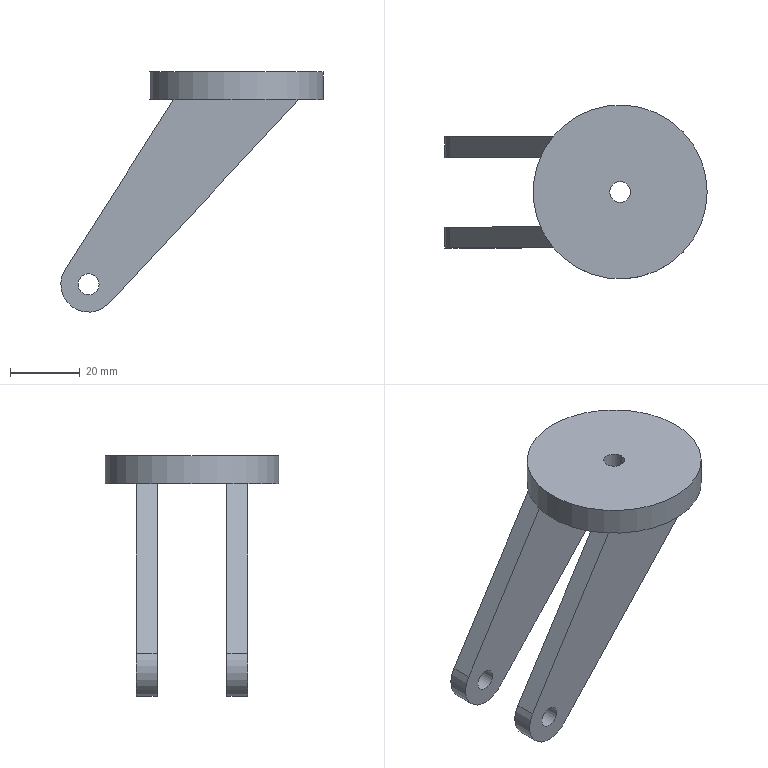Component | NX | UNI_WHEEL_CONN_FRAME | 1 solid | 16 faces | box 75.39 x 50 x 69.05 mm | volume 34354 mm3 | plane 10 | cylinder 6 | commonest cylinder face diameters 6 x3 16 x2 50 x1
STEP:
#1=CARTESIAN_POINT('',(0.,0.,0.));
#2=DIRECTION('',(0.,0.,1.));
#3=DIRECTION('',(1.,0.,0.));
#4=AXIS2_PLACEMENT_3D('',#1,#2,#3);
#5=CARTESIAN_POINT('',(447.437,-109.225,74.261));
#6=VERTEX_POINT('',#5);
#7=CARTESIAN_POINT('',(422.437,-109.225,74.261));
#8=DIRECTION('',(0.,0.,1.));
#9=DIRECTION('',(1.,0.,0.));
#10=AXIS2_PLACEMENT_3D('',#7,#8,#9);
#11=CIRCLE('',#10,25.);
#12=CARTESIAN_POINT('',(422.437,-109.225,74.261));
#13=DIRECTION('',(0.,0.,-1.));
#14=DIRECTION('',(-1.,0.,0.));
#15=AXIS2_PLACEMENT_3D('',#12,#13,#14);
#16=CYLINDRICAL_SURFACE('',#15,25.);
#17=CARTESIAN_POINT('',(9.425,0.));
#18=DIRECTION('',(-1.,0.));
#19=VECTOR('',#18,1.);
#20=LINE('',#17,#19);
#21=(GEOMETRIC_REPRESENTATION_CONTEXT(2)PARAMETRIC_REPRESENTATION_CONTEXT()REPRESENTATION_CONTEXT('',''));
#22=DEFINITIONAL_REPRESENTATION('',(#20),#21);
#23=PCURVE('',#16,#22);
#24=CARTESIAN_POINT('',(422.437,-109.225,74.261));
#25=DIRECTION('',(0.,0.,1.));
#26=DIRECTION('',(1.,0.,0.));
#27=AXIS2_PLACEMENT_3D('',#24,#25,#26);
#28=PLANE('',#27);
#29=CARTESIAN_POINT('',(0.,0.));
#30=DIRECTION('',(1.,0.));
#31=AXIS2_PLACEMENT_2D('',#29,#30);
#32=CIRCLE('',#31,25.);
#33=(GEOMETRIC_REPRESENTATION_CONTEXT(2)PARAMETRIC_REPRESENTATION_CONTEXT()REPRESENTATION_CONTEXT('',''));
#34=DEFINITIONAL_REPRESENTATION('',(#32),#33);
#35=PCURVE('',#28,#34);
#36=SURFACE_CURVE('',#11,(#23,#35),.PCURVE_S1.);
#37=EDGE_CURVE('',#6,#6,#36,.T.);
#38=ORIENTED_EDGE('',*,*,#37,.F.);
#39=CARTESIAN_POINT('',(447.437,-109.225,66.261));
#40=VERTEX_POINT('',#39);
#41=CARTESIAN_POINT('',(447.437,-109.225,74.261));
#42=CARTESIAN_POINT('',(447.437,-109.225,66.261));
#43=B_SPLINE_CURVE_WITH_KNOTS('',1,(#41,#42),.UNSPECIFIED.,.F.,.F.,(2,2),(0.,8.),.PIECEWISE_BEZIER_KNOTS.);
#44=CARTESIAN_POINT('',(9.425,0.));
#45=DIRECTION('',(0.,1.));
#46=VECTOR('',#45,1.);
#47=LINE('',#44,#46);
#48=(GEOMETRIC_REPRESENTATION_CONTEXT(2)PARAMETRIC_REPRESENTATION_CONTEXT()REPRESENTATION_CONTEXT('',''));
#49=DEFINITIONAL_REPRESENTATION('',(#47),#48);
#50=PCURVE('',#16,#49);
#51=CARTESIAN_POINT('',(3.142,0.));
#52=DIRECTION('',(0.,1.));
#53=VECTOR('',#52,1.);
#54=LINE('',#51,#53);
#55=(GEOMETRIC_REPRESENTATION_CONTEXT(2)PARAMETRIC_REPRESENTATION_CONTEXT()REPRESENTATION_CONTEXT('',''));
#56=DEFINITIONAL_REPRESENTATION('',(#54),#55);
#57=PCURVE('',#16,#56);
#58=SEAM_CURVE('',#43,(#50,#57),.PCURVE_S1.);
#59=EDGE_CURVE('',#6,#40,#58,.T.);
#60=ORIENTED_EDGE('',*,*,#59,.T.);
#61=CARTESIAN_POINT('',(422.437,-109.225,66.261));
#62=DIRECTION('',(0.,0.,1.));
#63=DIRECTION('',(1.,0.,0.));
#64=AXIS2_PLACEMENT_3D('',#61,#62,#63);
#65=CIRCLE('',#64,25.);
#66=CARTESIAN_POINT('',(9.425,8.));
#67=DIRECTION('',(-1.,0.));
#68=VECTOR('',#67,1.);
#69=LINE('',#66,#68);
#70=(GEOMETRIC_REPRESENTATION_CONTEXT(2)PARAMETRIC_REPRESENTATION_CONTEXT()REPRESENTATION_CONTEXT('',''));
#71=DEFINITIONAL_REPRESENTATION('',(#69),#70);
#72=PCURVE('',#16,#71);
#73=CARTESIAN_POINT('',(422.437,-109.225,66.261));
#74=DIRECTION('',(0.,0.,1.));
#75=DIRECTION('',(1.,0.,0.));
#76=AXIS2_PLACEMENT_3D('',#73,#74,#75);
#77=PLANE('',#76);
#78=CARTESIAN_POINT('',(0.,0.));
#79=DIRECTION('',(1.,0.));
#80=AXIS2_PLACEMENT_2D('',#78,#79);
#81=CIRCLE('',#80,25.);
#82=(GEOMETRIC_REPRESENTATION_CONTEXT(2)PARAMETRIC_REPRESENTATION_CONTEXT()REPRESENTATION_CONTEXT('',''));
#83=DEFINITIONAL_REPRESENTATION('',(#81),#82);
#84=PCURVE('',#77,#83);
#85=SURFACE_CURVE('',#65,(#72,#84),.PCURVE_S1.);
#86=EDGE_CURVE('',#40,#40,#85,.T.);
#87=ORIENTED_EDGE('',*,*,#86,.T.);
#88=ORIENTED_EDGE('',*,*,#59,.F.);
#89=EDGE_LOOP('',(#38,#60,#87,#88));
#90=FACE_BOUND('',#89,.T.);
#91=ADVANCED_FACE('',(#90),#16,.T.);
#92=CARTESIAN_POINT('',(425.437,-109.225,74.261));
#93=VERTEX_POINT('',#92);
#94=CARTESIAN_POINT('',(422.437,-109.225,74.261));
#95=DIRECTION('',(0.,0.,1.));
#96=DIRECTION('',(1.,0.,0.));
#97=AXIS2_PLACEMENT_3D('',#94,#95,#96);
#98=CIRCLE('',#97,3.);
#99=CARTESIAN_POINT('',(422.437,-109.225,74.261));
#100=DIRECTION('',(0.,0.,-1.));
#101=DIRECTION('',(-1.,0.,0.));
#102=AXIS2_PLACEMENT_3D('',#99,#100,#101);
#103=CYLINDRICAL_SURFACE('',#102,3.);
#104=CARTESIAN_POINT('',(9.425,0.));
#105=DIRECTION('',(-1.,0.));
#106=VECTOR('',#105,1.);
#107=LINE('',#104,#106);
#108=(GEOMETRIC_REPRESENTATION_CONTEXT(2)PARAMETRIC_REPRESENTATION_CONTEXT()REPRESENTATION_CONTEXT('',''));
#109=DEFINITIONAL_REPRESENTATION('',(#107),#108);
#110=PCURVE('',#103,#109);
#111=CARTESIAN_POINT('',(0.,0.));
#112=DIRECTION('',(1.,0.));
#113=AXIS2_PLACEMENT_2D('',#111,#112);
#114=CIRCLE('',#113,3.);
#115=(GEOMETRIC_REPRESENTATION_CONTEXT(2)PARAMETRIC_REPRESENTATION_CONTEXT()REPRESENTATION_CONTEXT('',''));
#116=DEFINITIONAL_REPRESENTATION('',(#114),#115);
#117=PCURVE('',#28,#116);
#118=SURFACE_CURVE('',#98,(#110,#117),.PCURVE_S1.);
#119=EDGE_CURVE('',#93,#93,#118,.T.);
#120=ORIENTED_EDGE('',*,*,#119,.F.);
#121=CARTESIAN_POINT('',(425.437,-109.225,66.261));
#122=VERTEX_POINT('',#121);
#123=CARTESIAN_POINT('',(425.437,-109.225,74.261));
#124=CARTESIAN_POINT('',(425.437,-109.225,66.261));
#125=B_SPLINE_CURVE_WITH_KNOTS('',1,(#123,#124),.UNSPECIFIED.,.F.,.F.,(2,2),(0.,8.),.PIECEWISE_BEZIER_KNOTS.);
#126=CARTESIAN_POINT('',(9.425,0.));
#127=DIRECTION('',(0.,1.));
#128=VECTOR('',#127,1.);
#129=LINE('',#126,#128);
#130=(GEOMETRIC_REPRESENTATION_CONTEXT(2)PARAMETRIC_REPRESENTATION_CONTEXT()REPRESENTATION_CONTEXT('',''));
#131=DEFINITIONAL_REPRESENTATION('',(#129),#130);
#132=PCURVE('',#103,#131);
#133=CARTESIAN_POINT('',(3.142,0.));
#134=DIRECTION('',(0.,1.));
#135=VECTOR('',#134,1.);
#136=LINE('',#133,#135);
#137=(GEOMETRIC_REPRESENTATION_CONTEXT(2)PARAMETRIC_REPRESENTATION_CONTEXT()REPRESENTATION_CONTEXT('',''));
#138=DEFINITIONAL_REPRESENTATION('',(#136),#137);
#139=PCURVE('',#103,#138);
#140=SEAM_CURVE('',#125,(#132,#139),.PCURVE_S1.);
#141=EDGE_CURVE('',#93,#122,#140,.T.);
#142=ORIENTED_EDGE('',*,*,#141,.T.);
#143=CARTESIAN_POINT('',(422.437,-109.225,66.261));
#144=DIRECTION('',(0.,0.,1.));
#145=DIRECTION('',(1.,0.,0.));
#146=AXIS2_PLACEMENT_3D('',#143,#144,#145);
#147=CIRCLE('',#146,3.);
#148=CARTESIAN_POINT('',(9.425,8.));
#149=DIRECTION('',(-1.,0.));
#150=VECTOR('',#149,1.);
#151=LINE('',#148,#150);
#152=(GEOMETRIC_REPRESENTATION_CONTEXT(2)PARAMETRIC_REPRESENTATION_CONTEXT()REPRESENTATION_CONTEXT('',''));
#153=DEFINITIONAL_REPRESENTATION('',(#151),#152);
#154=PCURVE('',#103,#153);
#155=CARTESIAN_POINT('',(0.,0.));
#156=DIRECTION('',(1.,0.));
#157=AXIS2_PLACEMENT_2D('',#155,#156);
#158=CIRCLE('',#157,3.);
#159=(GEOMETRIC_REPRESENTATION_CONTEXT(2)PARAMETRIC_REPRESENTATION_CONTEXT()REPRESENTATION_CONTEXT('',''));
#160=DEFINITIONAL_REPRESENTATION('',(#158),#159);
#161=PCURVE('',#77,#160);
#162=SURFACE_CURVE('',#147,(#154,#161),.PCURVE_S1.);
#163=EDGE_CURVE('',#122,#122,#162,.T.);
#164=ORIENTED_EDGE('',*,*,#163,.T.);
#165=ORIENTED_EDGE('',*,*,#141,.F.);
#166=EDGE_LOOP('',(#120,#142,#164,#165));
#167=FACE_BOUND('',#166,.F.);
#168=ADVANCED_FACE('',(#167),#103,.F.);
#169=ORIENTED_EDGE('',*,*,#37,.T.);
#170=EDGE_LOOP('',(#169));
#171=FACE_BOUND('',#170,.T.);
#172=ORIENTED_EDGE('',*,*,#119,.F.);
#173=EDGE_LOOP('',(#172));
#174=FACE_BOUND('',#173,.T.);
#175=ADVANCED_FACE('',(#171,#174),#28,.T.);
#176=CARTESIAN_POINT('',(440.437,-93.225,66.261));
#177=VERTEX_POINT('',#176);
#178=CARTESIAN_POINT('',(440.437,-99.225,66.261));
#179=VERTEX_POINT('',#178);
#180=CARTESIAN_POINT('',(440.437,-93.225,66.261));
#181=DIRECTION('',(0.,-1.,0.));
#182=VECTOR('',#181,1.);
#183=LINE('',#180,#182);
#184=CARTESIAN_POINT('',(18.,16.));
#185=DIRECTION('',(0.,-1.));
#186=VECTOR('',#185,1.);
#187=LINE('',#184,#186);
#188=(GEOMETRIC_REPRESENTATION_CONTEXT(2)PARAMETRIC_REPRESENTATION_CONTEXT()REPRESENTATION_CONTEXT('',''));
#189=DEFINITIONAL_REPRESENTATION('',(#187),#188);
#190=PCURVE('',#77,#189);
#191=CARTESIAN_POINT('',(385.896,-93.225,7.753));
#192=DIRECTION('',(0.7315,0.,-0.6819));
#193=DIRECTION('',(-0.6819,0.,-0.7315));
#194=AXIS2_PLACEMENT_3D('',#191,#192,#193);
#195=PLANE('',#194);
#196=CARTESIAN_POINT('',(-79.987,0.));
#197=DIRECTION('',(0.,-1.));
#198=VECTOR('',#197,1.);
#199=LINE('',#196,#198);
#200=(GEOMETRIC_REPRESENTATION_CONTEXT(2)PARAMETRIC_REPRESENTATION_CONTEXT()REPRESENTATION_CONTEXT('',''));
#201=DEFINITIONAL_REPRESENTATION('',(#199),#200);
#202=PCURVE('',#195,#201);
#203=SURFACE_CURVE('',#183,(#190,#202),.PCURVE_S1.);
#204=EDGE_CURVE('',#177,#179,#203,.T.);
#205=ORIENTED_EDGE('',*,*,#204,.F.);
#206=CARTESIAN_POINT('',(404.437,-93.225,66.261));
#207=VERTEX_POINT('',#206);
#208=CARTESIAN_POINT('',(440.437,-93.225,66.261));
#209=DIRECTION('',(-1.,0.,-0.));
#210=VECTOR('',#209,1.);
#211=LINE('',#208,#210);
#212=CARTESIAN_POINT('',(18.,16.));
#213=DIRECTION('',(-1.,0.));
#214=VECTOR('',#213,1.);
#215=LINE('',#212,#214);
#216=(GEOMETRIC_REPRESENTATION_CONTEXT(2)PARAMETRIC_REPRESENTATION_CONTEXT()REPRESENTATION_CONTEXT('',''));
#217=DEFINITIONAL_REPRESENTATION('',(#215),#216);
#218=PCURVE('',#77,#217);
#219=CARTESIAN_POINT('',(380.045,-93.225,13.208));
#220=DIRECTION('',(0.,-1.,0.));
#221=DIRECTION('',(0.,0.,-1.));
#222=AXIS2_PLACEMENT_3D('',#219,#220,#221);
#223=PLANE('',#222);
#224=CARTESIAN_POINT('',(-53.054,60.392));
#225=DIRECTION('',(0.,-1.));
#226=VECTOR('',#225,1.);
#227=LINE('',#224,#226);
#228=(GEOMETRIC_REPRESENTATION_CONTEXT(2)PARAMETRIC_REPRESENTATION_CONTEXT()REPRESENTATION_CONTEXT('',''));
#229=DEFINITIONAL_REPRESENTATION('',(#227),#228);
#230=PCURVE('',#223,#229);
#231=SURFACE_CURVE('',#211,(#218,#230),.PCURVE_S1.);
#232=EDGE_CURVE('',#177,#207,#231,.T.);
#233=ORIENTED_EDGE('',*,*,#232,.T.);
#234=CARTESIAN_POINT('',(404.437,-99.225,66.261));
#235=VERTEX_POINT('',#234);
#236=CARTESIAN_POINT('',(404.437,-93.225,66.261));
#237=DIRECTION('',(0.,-1.,0.));
#238=VECTOR('',#237,1.);
#239=LINE('',#236,#238);
#240=CARTESIAN_POINT('',(-18.,16.));
#241=DIRECTION('',(0.,-1.));
#242=VECTOR('',#241,1.);
#243=LINE('',#240,#242);
#244=(GEOMETRIC_REPRESENTATION_CONTEXT(2)PARAMETRIC_REPRESENTATION_CONTEXT()REPRESENTATION_CONTEXT('',''));
#245=DEFINITIONAL_REPRESENTATION('',(#243),#244);
#246=PCURVE('',#77,#245);
#247=CARTESIAN_POINT('',(404.437,-93.225,66.261));
#248=DIRECTION('',(-0.8428,0.,0.5383));
#249=DIRECTION('',(0.5383,0.,0.8428));
#250=AXIS2_PLACEMENT_3D('',#247,#248,#249);
#251=PLANE('',#250);
#252=CARTESIAN_POINT('',(0.,0.));
#253=DIRECTION('',(0.,-1.));
#254=VECTOR('',#253,1.);
#255=LINE('',#252,#254);
#256=(GEOMETRIC_REPRESENTATION_CONTEXT(2)PARAMETRIC_REPRESENTATION_CONTEXT()REPRESENTATION_CONTEXT('',''));
#257=DEFINITIONAL_REPRESENTATION('',(#255),#256);
#258=PCURVE('',#251,#257);
#259=SURFACE_CURVE('',#239,(#246,#258),.PCURVE_S1.);
#260=EDGE_CURVE('',#207,#235,#259,.T.);
#261=ORIENTED_EDGE('',*,*,#260,.T.);
#262=CARTESIAN_POINT('',(440.437,-99.225,66.261));
#263=DIRECTION('',(-1.,0.,-0.));
#264=VECTOR('',#263,1.);
#265=LINE('',#262,#264);
#266=CARTESIAN_POINT('',(18.,10.));
#267=DIRECTION('',(-1.,0.));
#268=VECTOR('',#267,1.);
#269=LINE('',#266,#268);
#270=(GEOMETRIC_REPRESENTATION_CONTEXT(2)PARAMETRIC_REPRESENTATION_CONTEXT()REPRESENTATION_CONTEXT('',''));
#271=DEFINITIONAL_REPRESENTATION('',(#269),#270);
#272=PCURVE('',#77,#271);
#273=CARTESIAN_POINT('',(380.045,-99.225,13.208));
#274=DIRECTION('',(0.,-1.,0.));
#275=DIRECTION('',(0.,0.,-1.));
#276=AXIS2_PLACEMENT_3D('',#273,#274,#275);
#277=PLANE('',#276);
#278=CARTESIAN_POINT('',(-53.054,60.392));
#279=DIRECTION('',(0.,-1.));
#280=VECTOR('',#279,1.);
#281=LINE('',#278,#280);
#282=(GEOMETRIC_REPRESENTATION_CONTEXT(2)PARAMETRIC_REPRESENTATION_CONTEXT()REPRESENTATION_CONTEXT('',''));
#283=DEFINITIONAL_REPRESENTATION('',(#281),#282);
#284=PCURVE('',#277,#283);
#285=SURFACE_CURVE('',#265,(#272,#284),.PCURVE_S1.);
#286=EDGE_CURVE('',#179,#235,#285,.T.);
#287=ORIENTED_EDGE('',*,*,#286,.F.);
#288=EDGE_LOOP('',(#205,#233,#261,#287));
#289=FACE_BOUND('',#288,.T.);
#290=CARTESIAN_POINT('',(440.437,-125.225,66.261));
#291=VERTEX_POINT('',#290);
#292=CARTESIAN_POINT('',(440.437,-119.225,66.261));
#293=VERTEX_POINT('',#292);
#294=CARTESIAN_POINT('',(440.437,-125.225,66.261));
#295=DIRECTION('',(0.,1.,0.));
#296=VECTOR('',#295,1.);
#297=LINE('',#294,#296);
#298=CARTESIAN_POINT('',(18.,-16.));
#299=DIRECTION('',(0.,1.));
#300=VECTOR('',#299,1.);
#301=LINE('',#298,#300);
#302=(GEOMETRIC_REPRESENTATION_CONTEXT(2)PARAMETRIC_REPRESENTATION_CONTEXT()REPRESENTATION_CONTEXT('',''));
#303=DEFINITIONAL_REPRESENTATION('',(#301),#302);
#304=PCURVE('',#77,#303);
#305=CARTESIAN_POINT('',(385.896,-125.225,7.753));
#306=DIRECTION('',(-0.7315,0.,0.6819));
#307=DIRECTION('',(0.6819,0.,0.7315));
#308=AXIS2_PLACEMENT_3D('',#305,#306,#307);
#309=PLANE('',#308);
#310=CARTESIAN_POINT('',(79.987,0.));
#311=DIRECTION('',(0.,1.));
#312=VECTOR('',#311,1.);
#313=LINE('',#310,#312);
#314=(GEOMETRIC_REPRESENTATION_CONTEXT(2)PARAMETRIC_REPRESENTATION_CONTEXT()REPRESENTATION_CONTEXT('',''));
#315=DEFINITIONAL_REPRESENTATION('',(#313),#314);
#316=PCURVE('',#309,#315);
#317=SURFACE_CURVE('',#297,(#304,#316),.PCURVE_S1.);
#318=EDGE_CURVE('',#291,#293,#317,.T.);
#319=ORIENTED_EDGE('',*,*,#318,.T.);
#320=CARTESIAN_POINT('',(404.437,-119.225,66.261));
#321=VERTEX_POINT('',#320);
#322=CARTESIAN_POINT('',(440.437,-119.225,66.261));
#323=DIRECTION('',(-1.,0.,-0.));
#324=VECTOR('',#323,1.);
#325=LINE('',#322,#324);
#326=CARTESIAN_POINT('',(18.,-10.));
#327=DIRECTION('',(-1.,0.));
#328=VECTOR('',#327,1.);
#329=LINE('',#326,#328);
#330=(GEOMETRIC_REPRESENTATION_CONTEXT(2)PARAMETRIC_REPRESENTATION_CONTEXT()REPRESENTATION_CONTEXT('',''));
#331=DEFINITIONAL_REPRESENTATION('',(#329),#330);
#332=PCURVE('',#77,#331);
#333=CARTESIAN_POINT('',(380.045,-119.225,13.208));
#334=DIRECTION('',(0.,-1.,0.));
#335=DIRECTION('',(0.,0.,-1.));
#336=AXIS2_PLACEMENT_3D('',#333,#334,#335);
#337=PLANE('',#336);
#338=CARTESIAN_POINT('',(-53.054,60.392));
#339=DIRECTION('',(0.,-1.));
#340=VECTOR('',#339,1.);
#341=LINE('',#338,#340);
#342=(GEOMETRIC_REPRESENTATION_CONTEXT(2)PARAMETRIC_REPRESENTATION_CONTEXT()REPRESENTATION_CONTEXT('',''));
#343=DEFINITIONAL_REPRESENTATION('',(#341),#342);
#344=PCURVE('',#337,#343);
#345=SURFACE_CURVE('',#325,(#332,#344),.PCURVE_S1.);
#346=EDGE_CURVE('',#293,#321,#345,.T.);
#347=ORIENTED_EDGE('',*,*,#346,.T.);
#348=CARTESIAN_POINT('',(404.437,-125.225,66.261));
#349=VERTEX_POINT('',#348);
#350=CARTESIAN_POINT('',(404.437,-125.225,66.261));
#351=DIRECTION('',(0.,1.,0.));
#352=VECTOR('',#351,1.);
#353=LINE('',#350,#352);
#354=CARTESIAN_POINT('',(-18.,-16.));
#355=DIRECTION('',(0.,1.));
#356=VECTOR('',#355,1.);
#357=LINE('',#354,#356);
#358=(GEOMETRIC_REPRESENTATION_CONTEXT(2)PARAMETRIC_REPRESENTATION_CONTEXT()REPRESENTATION_CONTEXT('',''));
#359=DEFINITIONAL_REPRESENTATION('',(#357),#358);
#360=PCURVE('',#77,#359);
#361=CARTESIAN_POINT('',(404.437,-125.225,66.261));
#362=DIRECTION('',(0.8428,0.,-0.5383));
#363=DIRECTION('',(-0.5383,0.,-0.8428));
#364=AXIS2_PLACEMENT_3D('',#361,#362,#363);
#365=PLANE('',#364);
#366=CARTESIAN_POINT('',(0.,0.));
#367=DIRECTION('',(0.,1.));
#368=VECTOR('',#367,1.);
#369=LINE('',#366,#368);
#370=(GEOMETRIC_REPRESENTATION_CONTEXT(2)PARAMETRIC_REPRESENTATION_CONTEXT()REPRESENTATION_CONTEXT('',''));
#371=DEFINITIONAL_REPRESENTATION('',(#369),#370);
#372=PCURVE('',#365,#371);
#373=SURFACE_CURVE('',#353,(#360,#372),.PCURVE_S1.);
#374=EDGE_CURVE('',#349,#321,#373,.T.);
#375=ORIENTED_EDGE('',*,*,#374,.F.);
#376=CARTESIAN_POINT('',(440.437,-125.225,66.261));
#377=DIRECTION('',(-1.,0.,-0.));
#378=VECTOR('',#377,1.);
#379=LINE('',#376,#378);
#380=CARTESIAN_POINT('',(18.,-16.));
#381=DIRECTION('',(-1.,0.));
#382=VECTOR('',#381,1.);
#383=LINE('',#380,#382);
#384=(GEOMETRIC_REPRESENTATION_CONTEXT(2)PARAMETRIC_REPRESENTATION_CONTEXT()REPRESENTATION_CONTEXT('',''));
#385=DEFINITIONAL_REPRESENTATION('',(#383),#384);
#386=PCURVE('',#77,#385);
#387=CARTESIAN_POINT('',(380.045,-125.225,13.208));
#388=DIRECTION('',(0.,-1.,0.));
#389=DIRECTION('',(0.,0.,-1.));
#390=AXIS2_PLACEMENT_3D('',#387,#388,#389);
#391=PLANE('',#390);
#392=CARTESIAN_POINT('',(-53.054,60.392));
#393=DIRECTION('',(0.,-1.));
#394=VECTOR('',#393,1.);
#395=LINE('',#392,#394);
#396=(GEOMETRIC_REPRESENTATION_CONTEXT(2)PARAMETRIC_REPRESENTATION_CONTEXT()REPRESENTATION_CONTEXT('',''));
#397=DEFINITIONAL_REPRESENTATION('',(#395),#396);
#398=PCURVE('',#391,#397);
#399=SURFACE_CURVE('',#379,(#386,#398),.PCURVE_S1.);
#400=EDGE_CURVE('',#291,#349,#399,.T.);
#401=ORIENTED_EDGE('',*,*,#400,.F.);
#402=EDGE_LOOP('',(#319,#347,#375,#401));
#403=FACE_BOUND('',#402,.T.);
#404=ORIENTED_EDGE('',*,*,#86,.F.);
#405=EDGE_LOOP('',(#404));
#406=FACE_BOUND('',#405,.T.);
#407=ORIENTED_EDGE('',*,*,#163,.T.);
#408=EDGE_LOOP('',(#407));
#409=FACE_BOUND('',#408,.T.);
#410=ADVANCED_FACE('',(#289,#403,#406,#409),#77,.F.);
#411=CARTESIAN_POINT('',(373.302,-119.225,17.514));
#412=VERTEX_POINT('',#411);
#413=CARTESIAN_POINT('',(385.896,-119.225,7.753));
#414=VERTEX_POINT('',#413);
#415=CARTESIAN_POINT('',(380.045,-119.225,13.208));
#416=DIRECTION('',(0.,-1.,0.));
#417=DIRECTION('',(1.,0.,0.));
#418=AXIS2_PLACEMENT_3D('',#415,#416,#417);
#419=CIRCLE('',#418,8.);
#420=CARTESIAN_POINT('',(380.045,-125.225,13.208));
#421=DIRECTION('',(0.,1.,0.));
#422=DIRECTION('',(0.,0.,1.));
#423=AXIS2_PLACEMENT_3D('',#420,#421,#422);
#424=CYLINDRICAL_SURFACE('',#423,8.);
#425=CARTESIAN_POINT('',(7.854,6.));
#426=DIRECTION('',(-1.,0.));
#427=VECTOR('',#426,1.);
#428=LINE('',#425,#427);
#429=(GEOMETRIC_REPRESENTATION_CONTEXT(2)PARAMETRIC_REPRESENTATION_CONTEXT()REPRESENTATION_CONTEXT('',''));
#430=DEFINITIONAL_REPRESENTATION('',(#428),#429);
#431=PCURVE('',#424,#430);
#432=CARTESIAN_POINT('',(0.,0.));
#433=DIRECTION('',(0.,1.));
#434=AXIS2_PLACEMENT_2D('',#432,#433);
#435=CIRCLE('',#434,8.);
#436=(GEOMETRIC_REPRESENTATION_CONTEXT(2)PARAMETRIC_REPRESENTATION_CONTEXT()REPRESENTATION_CONTEXT('',''));
#437=DEFINITIONAL_REPRESENTATION('',(#435),#436);
#438=PCURVE('',#337,#437);
#439=SURFACE_CURVE('',#419,(#431,#438),.PCURVE_S1.);
#440=EDGE_CURVE('',#412,#414,#439,.T.);
#441=ORIENTED_EDGE('',*,*,#440,.T.);
#442=CARTESIAN_POINT('',(385.896,-125.225,7.753));
#443=VERTEX_POINT('',#442);
#444=CARTESIAN_POINT('',(385.896,-125.225,7.753));
#445=DIRECTION('',(0.,1.,0.));
#446=VECTOR('',#445,1.);
#447=LINE('',#444,#446);
#448=CARTESIAN_POINT('',(2.321,0.));
#449=DIRECTION('',(0.,1.));
#450=VECTOR('',#449,1.);
#451=LINE('',#448,#450);
#452=(GEOMETRIC_REPRESENTATION_CONTEXT(2)PARAMETRIC_REPRESENTATION_CONTEXT()REPRESENTATION_CONTEXT('',''));
#453=DEFINITIONAL_REPRESENTATION('',(#451),#452);
#454=PCURVE('',#424,#453);
#455=CARTESIAN_POINT('',(-0.,0.));
#456=DIRECTION('',(0.,1.));
#457=VECTOR('',#456,1.);
#458=LINE('',#455,#457);
#459=(GEOMETRIC_REPRESENTATION_CONTEXT(2)PARAMETRIC_REPRESENTATION_CONTEXT()REPRESENTATION_CONTEXT('',''));
#460=DEFINITIONAL_REPRESENTATION('',(#458),#459);
#461=PCURVE('',#309,#460);
#462=SURFACE_CURVE('',#447,(#454,#461),.PCURVE_S1.);
#463=EDGE_CURVE('',#443,#414,#462,.T.);
#464=ORIENTED_EDGE('',*,*,#463,.F.);
#465=CARTESIAN_POINT('',(373.302,-125.225,17.514));
#466=VERTEX_POINT('',#465);
#467=CARTESIAN_POINT('',(380.045,-125.225,13.208));
#468=DIRECTION('',(0.,-1.,0.));
#469=DIRECTION('',(1.,0.,0.));
#470=AXIS2_PLACEMENT_3D('',#467,#468,#469);
#471=CIRCLE('',#470,8.);
#472=CARTESIAN_POINT('',(7.854,0.));
#473=DIRECTION('',(-1.,0.));
#474=VECTOR('',#473,1.);
#475=LINE('',#472,#474);
#476=(GEOMETRIC_REPRESENTATION_CONTEXT(2)PARAMETRIC_REPRESENTATION_CONTEXT()REPRESENTATION_CONTEXT('',''));
#477=DEFINITIONAL_REPRESENTATION('',(#475),#476);
#478=PCURVE('',#424,#477);
#479=CARTESIAN_POINT('',(0.,0.));
#480=DIRECTION('',(0.,1.));
#481=AXIS2_PLACEMENT_2D('',#479,#480);
#482=CIRCLE('',#481,8.);
#483=(GEOMETRIC_REPRESENTATION_CONTEXT(2)PARAMETRIC_REPRESENTATION_CONTEXT()REPRESENTATION_CONTEXT('',''));
#484=DEFINITIONAL_REPRESENTATION('',(#482),#483);
#485=PCURVE('',#391,#484);
#486=SURFACE_CURVE('',#471,(#478,#485),.PCURVE_S1.);
#487=EDGE_CURVE('',#466,#443,#486,.T.);
#488=ORIENTED_EDGE('',*,*,#487,.F.);
#489=CARTESIAN_POINT('',(373.302,-125.225,17.514));
#490=DIRECTION('',(0.,1.,0.));
#491=VECTOR('',#490,1.);
#492=LINE('',#489,#491);
#493=CARTESIAN_POINT('',(5.281,0.));
#494=DIRECTION('',(0.,1.));
#495=VECTOR('',#494,1.);
#496=LINE('',#493,#495);
#497=(GEOMETRIC_REPRESENTATION_CONTEXT(2)PARAMETRIC_REPRESENTATION_CONTEXT()REPRESENTATION_CONTEXT('',''));
#498=DEFINITIONAL_REPRESENTATION('',(#496),#497);
#499=PCURVE('',#424,#498);
#500=CARTESIAN_POINT('',(57.842,0.));
#501=DIRECTION('',(0.,1.));
#502=VECTOR('',#501,1.);
#503=LINE('',#500,#502);
#504=(GEOMETRIC_REPRESENTATION_CONTEXT(2)PARAMETRIC_REPRESENTATION_CONTEXT()REPRESENTATION_CONTEXT('',''));
#505=DEFINITIONAL_REPRESENTATION('',(#503),#504);
#506=PCURVE('',#365,#505);
#507=SURFACE_CURVE('',#492,(#499,#506),.PCURVE_S1.);
#508=EDGE_CURVE('',#466,#412,#507,.T.);
#509=ORIENTED_EDGE('',*,*,#508,.T.);
#510=EDGE_LOOP('',(#441,#464,#488,#509));
#511=FACE_BOUND('',#510,.T.);
#512=ADVANCED_FACE('',(#511),#424,.T.);
#513=CARTESIAN_POINT('',(385.896,-119.225,7.753));
#514=DIRECTION('',(0.6819,0.,0.7315));
#515=VECTOR('',#514,1.);
#516=LINE('',#513,#515);
#517=CARTESIAN_POINT('',(0.,6.));
#518=DIRECTION('',(1.,0.));
#519=VECTOR('',#518,1.);
#520=LINE('',#517,#519);
#521=(GEOMETRIC_REPRESENTATION_CONTEXT(2)PARAMETRIC_REPRESENTATION_CONTEXT()REPRESENTATION_CONTEXT('',''));
#522=DEFINITIONAL_REPRESENTATION('',(#520),#521);
#523=PCURVE('',#309,#522);
#524=CARTESIAN_POINT('',(5.455,5.852));
#525=DIRECTION('',(-0.7315,0.6819));
#526=VECTOR('',#525,1.);
#527=LINE('',#524,#526);
#528=(GEOMETRIC_REPRESENTATION_CONTEXT(2)PARAMETRIC_REPRESENTATION_CONTEXT()REPRESENTATION_CONTEXT('',''));
#529=DEFINITIONAL_REPRESENTATION('',(#527),#528);
#530=PCURVE('',#337,#529);
#531=SURFACE_CURVE('',#516,(#523,#530),.PCURVE_S1.);
#532=EDGE_CURVE('',#414,#293,#531,.T.);
#533=ORIENTED_EDGE('',*,*,#532,.T.);
#534=ORIENTED_EDGE('',*,*,#318,.F.);
#535=CARTESIAN_POINT('',(385.896,-125.225,7.753));
#536=DIRECTION('',(0.6819,0.,0.7315));
#537=VECTOR('',#536,1.);
#538=LINE('',#535,#537);
#539=CARTESIAN_POINT('',(0.,0.));
#540=DIRECTION('',(1.,0.));
#541=VECTOR('',#540,1.);
#542=LINE('',#539,#541);
#543=(GEOMETRIC_REPRESENTATION_CONTEXT(2)PARAMETRIC_REPRESENTATION_CONTEXT()REPRESENTATION_CONTEXT('',''));
#544=DEFINITIONAL_REPRESENTATION('',(#542),#543);
#545=PCURVE('',#309,#544);
#546=CARTESIAN_POINT('',(5.455,5.852));
#547=DIRECTION('',(-0.7315,0.6819));
#548=VECTOR('',#547,1.);
#549=LINE('',#546,#548);
#550=(GEOMETRIC_REPRESENTATION_CONTEXT(2)PARAMETRIC_REPRESENTATION_CONTEXT()REPRESENTATION_CONTEXT('',''));
#551=DEFINITIONAL_REPRESENTATION('',(#549),#550);
#552=PCURVE('',#391,#551);
#553=SURFACE_CURVE('',#538,(#545,#552),.PCURVE_S1.);
#554=EDGE_CURVE('',#443,#291,#553,.T.);
#555=ORIENTED_EDGE('',*,*,#554,.F.);
#556=ORIENTED_EDGE('',*,*,#463,.T.);
#557=EDGE_LOOP('',(#533,#534,#555,#556));
#558=FACE_BOUND('',#557,.T.);
#559=ADVANCED_FACE('',(#558),#309,.F.);
#560=CARTESIAN_POINT('',(404.437,-119.225,66.261));
#561=DIRECTION('',(-0.5383,0.,-0.8428));
#562=VECTOR('',#561,1.);
#563=LINE('',#560,#562);
#564=CARTESIAN_POINT('',(0.,6.));
#565=DIRECTION('',(1.,0.));
#566=VECTOR('',#565,1.);
#567=LINE('',#564,#566);
#568=(GEOMETRIC_REPRESENTATION_CONTEXT(2)PARAMETRIC_REPRESENTATION_CONTEXT()REPRESENTATION_CONTEXT('',''));
#569=DEFINITIONAL_REPRESENTATION('',(#567),#568);
#570=PCURVE('',#365,#569);
#571=CARTESIAN_POINT('',(-53.054,24.392));
#572=DIRECTION('',(0.8428,-0.5383));
#573=VECTOR('',#572,1.);
#574=LINE('',#571,#573);
#575=(GEOMETRIC_REPRESENTATION_CONTEXT(2)PARAMETRIC_REPRESENTATION_CONTEXT()REPRESENTATION_CONTEXT('',''));
#576=DEFINITIONAL_REPRESENTATION('',(#574),#575);
#577=PCURVE('',#337,#576);
#578=SURFACE_CURVE('',#563,(#570,#577),.PCURVE_S1.);
#579=EDGE_CURVE('',#321,#412,#578,.T.);
#580=ORIENTED_EDGE('',*,*,#579,.T.);
#581=ORIENTED_EDGE('',*,*,#508,.F.);
#582=CARTESIAN_POINT('',(404.437,-125.225,66.261));
#583=DIRECTION('',(-0.5383,0.,-0.8428));
#584=VECTOR('',#583,1.);
#585=LINE('',#582,#584);
#586=CARTESIAN_POINT('',(0.,0.));
#587=DIRECTION('',(1.,0.));
#588=VECTOR('',#587,1.);
#589=LINE('',#586,#588);
#590=(GEOMETRIC_REPRESENTATION_CONTEXT(2)PARAMETRIC_REPRESENTATION_CONTEXT()REPRESENTATION_CONTEXT('',''));
#591=DEFINITIONAL_REPRESENTATION('',(#589),#590);
#592=PCURVE('',#365,#591);
#593=CARTESIAN_POINT('',(-53.054,24.392));
#594=DIRECTION('',(0.8428,-0.5383));
#595=VECTOR('',#594,1.);
#596=LINE('',#593,#595);
#597=(GEOMETRIC_REPRESENTATION_CONTEXT(2)PARAMETRIC_REPRESENTATION_CONTEXT()REPRESENTATION_CONTEXT('',''));
#598=DEFINITIONAL_REPRESENTATION('',(#596),#597);
#599=PCURVE('',#391,#598);
#600=SURFACE_CURVE('',#585,(#592,#599),.PCURVE_S1.);
#601=EDGE_CURVE('',#349,#466,#600,.T.);
#602=ORIENTED_EDGE('',*,*,#601,.F.);
#603=ORIENTED_EDGE('',*,*,#374,.T.);
#604=EDGE_LOOP('',(#580,#581,#602,#603));
#605=FACE_BOUND('',#604,.T.);
#606=ADVANCED_FACE('',(#605),#365,.F.);
#607=CARTESIAN_POINT('',(383.045,-125.225,13.208));
#608=VERTEX_POINT('',#607);
#609=CARTESIAN_POINT('',(380.045,-125.225,13.208));
#610=DIRECTION('',(0.,-1.,0.));
#611=DIRECTION('',(1.,0.,0.));
#612=AXIS2_PLACEMENT_3D('',#609,#610,#611);
#613=CIRCLE('',#612,3.);
#614=CARTESIAN_POINT('',(380.045,-125.225,13.208));
#615=DIRECTION('',(0.,1.,0.));
#616=DIRECTION('',(0.,0.,1.));
#617=AXIS2_PLACEMENT_3D('',#614,#615,#616);
#618=CYLINDRICAL_SURFACE('',#617,3.);
#619=CARTESIAN_POINT('',(7.854,0.));
#620=DIRECTION('',(-1.,0.));
#621=VECTOR('',#620,1.);
#622=LINE('',#619,#621);
#623=(GEOMETRIC_REPRESENTATION_CONTEXT(2)PARAMETRIC_REPRESENTATION_CONTEXT()REPRESENTATION_CONTEXT('',''));
#624=DEFINITIONAL_REPRESENTATION('',(#622),#623);
#625=PCURVE('',#618,#624);
#626=CARTESIAN_POINT('',(0.,0.));
#627=DIRECTION('',(0.,1.));
#628=AXIS2_PLACEMENT_2D('',#626,#627);
#629=CIRCLE('',#628,3.);
#630=(GEOMETRIC_REPRESENTATION_CONTEXT(2)PARAMETRIC_REPRESENTATION_CONTEXT()REPRESENTATION_CONTEXT('',''));
#631=DEFINITIONAL_REPRESENTATION('',(#629),#630);
#632=PCURVE('',#391,#631);
#633=SURFACE_CURVE('',#613,(#625,#632),.PCURVE_S1.);
#634=EDGE_CURVE('',#608,#608,#633,.T.);
#635=ORIENTED_EDGE('',*,*,#634,.F.);
#636=CARTESIAN_POINT('',(383.045,-119.225,13.208));
#637=VERTEX_POINT('',#636);
#638=CARTESIAN_POINT('',(383.045,-125.225,13.208));
#639=CARTESIAN_POINT('',(383.045,-119.225,13.208));
#640=B_SPLINE_CURVE_WITH_KNOTS('',1,(#638,#639),.UNSPECIFIED.,.F.,.F.,(2,2),(0.,6.),.PIECEWISE_BEZIER_KNOTS.);
#641=CARTESIAN_POINT('',(7.854,0.));
#642=DIRECTION('',(0.,1.));
#643=VECTOR('',#642,1.);
#644=LINE('',#641,#643);
#645=(GEOMETRIC_REPRESENTATION_CONTEXT(2)PARAMETRIC_REPRESENTATION_CONTEXT()REPRESENTATION_CONTEXT('',''));
#646=DEFINITIONAL_REPRESENTATION('',(#644),#645);
#647=PCURVE('',#618,#646);
#648=CARTESIAN_POINT('',(1.571,0.));
#649=DIRECTION('',(0.,1.));
#650=VECTOR('',#649,1.);
#651=LINE('',#648,#650);
#652=(GEOMETRIC_REPRESENTATION_CONTEXT(2)PARAMETRIC_REPRESENTATION_CONTEXT()REPRESENTATION_CONTEXT('',''));
#653=DEFINITIONAL_REPRESENTATION('',(#651),#652);
#654=PCURVE('',#618,#653);
#655=SEAM_CURVE('',#640,(#647,#654),.PCURVE_S1.);
#656=EDGE_CURVE('',#608,#637,#655,.T.);
#657=ORIENTED_EDGE('',*,*,#656,.T.);
#658=CARTESIAN_POINT('',(380.045,-119.225,13.208));
#659=DIRECTION('',(0.,-1.,0.));
#660=DIRECTION('',(1.,0.,0.));
#661=AXIS2_PLACEMENT_3D('',#658,#659,#660);
#662=CIRCLE('',#661,3.);
#663=CARTESIAN_POINT('',(7.854,6.));
#664=DIRECTION('',(-1.,0.));
#665=VECTOR('',#664,1.);
#666=LINE('',#663,#665);
#667=(GEOMETRIC_REPRESENTATION_CONTEXT(2)PARAMETRIC_REPRESENTATION_CONTEXT()REPRESENTATION_CONTEXT('',''));
#668=DEFINITIONAL_REPRESENTATION('',(#666),#667);
#669=PCURVE('',#618,#668);
#670=CARTESIAN_POINT('',(0.,0.));
#671=DIRECTION('',(0.,1.));
#672=AXIS2_PLACEMENT_2D('',#670,#671);
#673=CIRCLE('',#672,3.);
#674=(GEOMETRIC_REPRESENTATION_CONTEXT(2)PARAMETRIC_REPRESENTATION_CONTEXT()REPRESENTATION_CONTEXT('',''));
#675=DEFINITIONAL_REPRESENTATION('',(#673),#674);
#676=PCURVE('',#337,#675);
#677=SURFACE_CURVE('',#662,(#669,#676),.PCURVE_S1.);
#678=EDGE_CURVE('',#637,#637,#677,.T.);
#679=ORIENTED_EDGE('',*,*,#678,.T.);
#680=ORIENTED_EDGE('',*,*,#656,.F.);
#681=EDGE_LOOP('',(#635,#657,#679,#680));
#682=FACE_BOUND('',#681,.F.);
#683=ADVANCED_FACE('',(#682),#618,.F.);
#684=ORIENTED_EDGE('',*,*,#487,.T.);
#685=ORIENTED_EDGE('',*,*,#554,.T.);
#686=ORIENTED_EDGE('',*,*,#400,.T.);
#687=ORIENTED_EDGE('',*,*,#601,.T.);
#688=EDGE_LOOP('',(#684,#685,#686,#687));
#689=FACE_BOUND('',#688,.T.);
#690=ORIENTED_EDGE('',*,*,#634,.F.);
#691=EDGE_LOOP('',(#690));
#692=FACE_BOUND('',#691,.T.);
#693=ADVANCED_FACE('',(#689,#692),#391,.T.);
#694=ORIENTED_EDGE('',*,*,#440,.F.);
#695=ORIENTED_EDGE('',*,*,#579,.F.);
#696=ORIENTED_EDGE('',*,*,#346,.F.);
#697=ORIENTED_EDGE('',*,*,#532,.F.);
#698=EDGE_LOOP('',(#694,#695,#696,#697));
#699=FACE_BOUND('',#698,.T.);
#700=ORIENTED_EDGE('',*,*,#678,.T.);
#701=EDGE_LOOP('',(#700));
#702=FACE_BOUND('',#701,.T.);
#703=ADVANCED_FACE('',(#699,#702),#337,.F.);
#704=CARTESIAN_POINT('',(373.302,-99.225,17.514));
#705=VERTEX_POINT('',#704);
#706=CARTESIAN_POINT('',(385.896,-99.225,7.753));
#707=VERTEX_POINT('',#706);
#708=CARTESIAN_POINT('',(380.045,-99.225,13.208));
#709=DIRECTION('',(0.,-1.,0.));
#710=DIRECTION('',(1.,0.,0.));
#711=AXIS2_PLACEMENT_3D('',#708,#709,#710);
#712=CIRCLE('',#711,8.);
#713=CARTESIAN_POINT('',(380.045,-93.225,13.208));
#714=DIRECTION('',(0.,-1.,0.));
#715=DIRECTION('',(0.,0.,-1.));
#716=AXIS2_PLACEMENT_3D('',#713,#714,#715);
#717=CYLINDRICAL_SURFACE('',#716,8.);
#718=CARTESIAN_POINT('',(1.571,6.));
#719=DIRECTION('',(1.,0.));
#720=VECTOR('',#719,1.);
#721=LINE('',#718,#720);
#722=(GEOMETRIC_REPRESENTATION_CONTEXT(2)PARAMETRIC_REPRESENTATION_CONTEXT()REPRESENTATION_CONTEXT('',''));
#723=DEFINITIONAL_REPRESENTATION('',(#721),#722);
#724=PCURVE('',#717,#723);
#725=CARTESIAN_POINT('',(0.,0.));
#726=DIRECTION('',(0.,1.));
#727=AXIS2_PLACEMENT_2D('',#725,#726);
#728=CIRCLE('',#727,8.);
#729=(GEOMETRIC_REPRESENTATION_CONTEXT(2)PARAMETRIC_REPRESENTATION_CONTEXT()REPRESENTATION_CONTEXT('',''));
#730=DEFINITIONAL_REPRESENTATION('',(#728),#729);
#731=PCURVE('',#277,#730);
#732=SURFACE_CURVE('',#712,(#724,#731),.PCURVE_S1.);
#733=EDGE_CURVE('',#705,#707,#732,.T.);
#734=ORIENTED_EDGE('',*,*,#733,.F.);
#735=CARTESIAN_POINT('',(373.302,-93.225,17.514));
#736=VERTEX_POINT('',#735);
#737=CARTESIAN_POINT('',(373.302,-93.225,17.514));
#738=DIRECTION('',(0.,-1.,0.));
#739=VECTOR('',#738,1.);
#740=LINE('',#737,#739);
#741=CARTESIAN_POINT('',(4.144,0.));
#742=DIRECTION('',(0.,1.));
#743=VECTOR('',#742,1.);
#744=LINE('',#741,#743);
#745=(GEOMETRIC_REPRESENTATION_CONTEXT(2)PARAMETRIC_REPRESENTATION_CONTEXT()REPRESENTATION_CONTEXT('',''));
#746=DEFINITIONAL_REPRESENTATION('',(#744),#745);
#747=PCURVE('',#717,#746);
#748=CARTESIAN_POINT('',(-57.842,0.));
#749=DIRECTION('',(0.,-1.));
#750=VECTOR('',#749,1.);
#751=LINE('',#748,#750);
#752=(GEOMETRIC_REPRESENTATION_CONTEXT(2)PARAMETRIC_REPRESENTATION_CONTEXT()REPRESENTATION_CONTEXT('',''));
#753=DEFINITIONAL_REPRESENTATION('',(#751),#752);
#754=PCURVE('',#251,#753);
#755=SURFACE_CURVE('',#740,(#747,#754),.PCURVE_S1.);
#756=EDGE_CURVE('',#736,#705,#755,.T.);
#757=ORIENTED_EDGE('',*,*,#756,.F.);
#758=CARTESIAN_POINT('',(385.896,-93.225,7.753));
#759=VERTEX_POINT('',#758);
#760=CARTESIAN_POINT('',(380.045,-93.225,13.208));
#761=DIRECTION('',(0.,-1.,0.));
#762=DIRECTION('',(1.,0.,0.));
#763=AXIS2_PLACEMENT_3D('',#760,#761,#762);
#764=CIRCLE('',#763,8.);
#765=CARTESIAN_POINT('',(1.571,0.));
#766=DIRECTION('',(1.,0.));
#767=VECTOR('',#766,1.);
#768=LINE('',#765,#767);
#769=(GEOMETRIC_REPRESENTATION_CONTEXT(2)PARAMETRIC_REPRESENTATION_CONTEXT()REPRESENTATION_CONTEXT('',''));
#770=DEFINITIONAL_REPRESENTATION('',(#768),#769);
#771=PCURVE('',#717,#770);
#772=CARTESIAN_POINT('',(0.,0.));
#773=DIRECTION('',(0.,1.));
#774=AXIS2_PLACEMENT_2D('',#772,#773);
#775=CIRCLE('',#774,8.);
#776=(GEOMETRIC_REPRESENTATION_CONTEXT(2)PARAMETRIC_REPRESENTATION_CONTEXT()REPRESENTATION_CONTEXT('',''));
#777=DEFINITIONAL_REPRESENTATION('',(#775),#776);
#778=PCURVE('',#223,#777);
#779=SURFACE_CURVE('',#764,(#771,#778),.PCURVE_S1.);
#780=EDGE_CURVE('',#736,#759,#779,.T.);
#781=ORIENTED_EDGE('',*,*,#780,.T.);
#782=CARTESIAN_POINT('',(385.896,-93.225,7.753));
#783=DIRECTION('',(0.,-1.,0.));
#784=VECTOR('',#783,1.);
#785=LINE('',#782,#784);
#786=CARTESIAN_POINT('',(7.104,0.));
#787=DIRECTION('',(0.,1.));
#788=VECTOR('',#787,1.);
#789=LINE('',#786,#788);
#790=(GEOMETRIC_REPRESENTATION_CONTEXT(2)PARAMETRIC_REPRESENTATION_CONTEXT()REPRESENTATION_CONTEXT('',''));
#791=DEFINITIONAL_REPRESENTATION('',(#789),#790);
#792=PCURVE('',#717,#791);
#793=CARTESIAN_POINT('',(0.,0.));
#794=DIRECTION('',(0.,-1.));
#795=VECTOR('',#794,1.);
#796=LINE('',#793,#795);
#797=(GEOMETRIC_REPRESENTATION_CONTEXT(2)PARAMETRIC_REPRESENTATION_CONTEXT()REPRESENTATION_CONTEXT('',''));
#798=DEFINITIONAL_REPRESENTATION('',(#796),#797);
#799=PCURVE('',#195,#798);
#800=SURFACE_CURVE('',#785,(#792,#799),.PCURVE_S1.);
#801=EDGE_CURVE('',#759,#707,#800,.T.);
#802=ORIENTED_EDGE('',*,*,#801,.T.);
#803=EDGE_LOOP('',(#734,#757,#781,#802));
#804=FACE_BOUND('',#803,.T.);
#805=ADVANCED_FACE('',(#804),#717,.T.);
#806=CARTESIAN_POINT('',(385.896,-99.225,7.753));
#807=DIRECTION('',(0.6819,0.,0.7315));
#808=VECTOR('',#807,1.);
#809=LINE('',#806,#808);
#810=CARTESIAN_POINT('',(0.,-6.));
#811=DIRECTION('',(-1.,0.));
#812=VECTOR('',#811,1.);
#813=LINE('',#810,#812);
#814=(GEOMETRIC_REPRESENTATION_CONTEXT(2)PARAMETRIC_REPRESENTATION_CONTEXT()REPRESENTATION_CONTEXT('',''));
#815=DEFINITIONAL_REPRESENTATION('',(#813),#814);
#816=PCURVE('',#195,#815);
#817=CARTESIAN_POINT('',(5.455,5.852));
#818=DIRECTION('',(-0.7315,0.6819));
#819=VECTOR('',#818,1.);
#820=LINE('',#817,#819);
#821=(GEOMETRIC_REPRESENTATION_CONTEXT(2)PARAMETRIC_REPRESENTATION_CONTEXT()REPRESENTATION_CONTEXT('',''));
#822=DEFINITIONAL_REPRESENTATION('',(#820),#821);
#823=PCURVE('',#277,#822);
#824=SURFACE_CURVE('',#809,(#816,#823),.PCURVE_S1.);
#825=EDGE_CURVE('',#707,#179,#824,.T.);
#826=ORIENTED_EDGE('',*,*,#825,.F.);
#827=ORIENTED_EDGE('',*,*,#801,.F.);
#828=CARTESIAN_POINT('',(385.896,-93.225,7.753));
#829=DIRECTION('',(0.6819,0.,0.7315));
#830=VECTOR('',#829,1.);
#831=LINE('',#828,#830);
#832=CARTESIAN_POINT('',(0.,0.));
#833=DIRECTION('',(-1.,0.));
#834=VECTOR('',#833,1.);
#835=LINE('',#832,#834);
#836=(GEOMETRIC_REPRESENTATION_CONTEXT(2)PARAMETRIC_REPRESENTATION_CONTEXT()REPRESENTATION_CONTEXT('',''));
#837=DEFINITIONAL_REPRESENTATION('',(#835),#836);
#838=PCURVE('',#195,#837);
#839=CARTESIAN_POINT('',(5.455,5.852));
#840=DIRECTION('',(-0.7315,0.6819));
#841=VECTOR('',#840,1.);
#842=LINE('',#839,#841);
#843=(GEOMETRIC_REPRESENTATION_CONTEXT(2)PARAMETRIC_REPRESENTATION_CONTEXT()REPRESENTATION_CONTEXT('',''));
#844=DEFINITIONAL_REPRESENTATION('',(#842),#843);
#845=PCURVE('',#223,#844);
#846=SURFACE_CURVE('',#831,(#838,#845),.PCURVE_S1.);
#847=EDGE_CURVE('',#759,#177,#846,.T.);
#848=ORIENTED_EDGE('',*,*,#847,.T.);
#849=ORIENTED_EDGE('',*,*,#204,.T.);
#850=EDGE_LOOP('',(#826,#827,#848,#849));
#851=FACE_BOUND('',#850,.T.);
#852=ADVANCED_FACE('',(#851),#195,.T.);
#853=CARTESIAN_POINT('',(404.437,-99.225,66.261));
#854=DIRECTION('',(-0.5383,0.,-0.8428));
#855=VECTOR('',#854,1.);
#856=LINE('',#853,#855);
#857=CARTESIAN_POINT('',(0.,-6.));
#858=DIRECTION('',(-1.,0.));
#859=VECTOR('',#858,1.);
#860=LINE('',#857,#859);
#861=(GEOMETRIC_REPRESENTATION_CONTEXT(2)PARAMETRIC_REPRESENTATION_CONTEXT()REPRESENTATION_CONTEXT('',''));
#862=DEFINITIONAL_REPRESENTATION('',(#860),#861);
#863=PCURVE('',#251,#862);
#864=CARTESIAN_POINT('',(-53.054,24.392));
#865=DIRECTION('',(0.8428,-0.5383));
#866=VECTOR('',#865,1.);
#867=LINE('',#864,#866);
#868=(GEOMETRIC_REPRESENTATION_CONTEXT(2)PARAMETRIC_REPRESENTATION_CONTEXT()REPRESENTATION_CONTEXT('',''));
#869=DEFINITIONAL_REPRESENTATION('',(#867),#868);
#870=PCURVE('',#277,#869);
#871=SURFACE_CURVE('',#856,(#863,#870),.PCURVE_S1.);
#872=EDGE_CURVE('',#235,#705,#871,.T.);
#873=ORIENTED_EDGE('',*,*,#872,.F.);
#874=ORIENTED_EDGE('',*,*,#260,.F.);
#875=CARTESIAN_POINT('',(404.437,-93.225,66.261));
#876=DIRECTION('',(-0.5383,0.,-0.8428));
#877=VECTOR('',#876,1.);
#878=LINE('',#875,#877);
#879=CARTESIAN_POINT('',(0.,0.));
#880=DIRECTION('',(-1.,0.));
#881=VECTOR('',#880,1.);
#882=LINE('',#879,#881);
#883=(GEOMETRIC_REPRESENTATION_CONTEXT(2)PARAMETRIC_REPRESENTATION_CONTEXT()REPRESENTATION_CONTEXT('',''));
#884=DEFINITIONAL_REPRESENTATION('',(#882),#883);
#885=PCURVE('',#251,#884);
#886=CARTESIAN_POINT('',(-53.054,24.392));
#887=DIRECTION('',(0.8428,-0.5383));
#888=VECTOR('',#887,1.);
#889=LINE('',#886,#888);
#890=(GEOMETRIC_REPRESENTATION_CONTEXT(2)PARAMETRIC_REPRESENTATION_CONTEXT()REPRESENTATION_CONTEXT('',''));
#891=DEFINITIONAL_REPRESENTATION('',(#889),#890);
#892=PCURVE('',#223,#891);
#893=SURFACE_CURVE('',#878,(#885,#892),.PCURVE_S1.);
#894=EDGE_CURVE('',#207,#736,#893,.T.);
#895=ORIENTED_EDGE('',*,*,#894,.T.);
#896=ORIENTED_EDGE('',*,*,#756,.T.);
#897=EDGE_LOOP('',(#873,#874,#895,#896));
#898=FACE_BOUND('',#897,.T.);
#899=ADVANCED_FACE('',(#898),#251,.T.);
#900=CARTESIAN_POINT('',(383.045,-93.225,13.208));
#901=VERTEX_POINT('',#900);
#902=CARTESIAN_POINT('',(380.045,-93.225,13.208));
#903=DIRECTION('',(0.,-1.,0.));
#904=DIRECTION('',(1.,0.,0.));
#905=AXIS2_PLACEMENT_3D('',#902,#903,#904);
#906=CIRCLE('',#905,3.);
#907=CARTESIAN_POINT('',(380.045,-93.225,13.208));
#908=DIRECTION('',(0.,-1.,0.));
#909=DIRECTION('',(0.,0.,-1.));
#910=AXIS2_PLACEMENT_3D('',#907,#908,#909);
#911=CYLINDRICAL_SURFACE('',#910,3.);
#912=CARTESIAN_POINT('',(1.571,0.));
#913=DIRECTION('',(1.,0.));
#914=VECTOR('',#913,1.);
#915=LINE('',#912,#914);
#916=(GEOMETRIC_REPRESENTATION_CONTEXT(2)PARAMETRIC_REPRESENTATION_CONTEXT()REPRESENTATION_CONTEXT('',''));
#917=DEFINITIONAL_REPRESENTATION('',(#915),#916);
#918=PCURVE('',#911,#917);
#919=CARTESIAN_POINT('',(0.,0.));
#920=DIRECTION('',(0.,1.));
#921=AXIS2_PLACEMENT_2D('',#919,#920);
#922=CIRCLE('',#921,3.);
#923=(GEOMETRIC_REPRESENTATION_CONTEXT(2)PARAMETRIC_REPRESENTATION_CONTEXT()REPRESENTATION_CONTEXT('',''));
#924=DEFINITIONAL_REPRESENTATION('',(#922),#923);
#925=PCURVE('',#223,#924);
#926=SURFACE_CURVE('',#906,(#918,#925),.PCURVE_S1.);
#927=EDGE_CURVE('',#901,#901,#926,.T.);
#928=ORIENTED_EDGE('',*,*,#927,.T.);
#929=CARTESIAN_POINT('',(383.045,-99.225,13.208));
#930=VERTEX_POINT('',#929);
#931=CARTESIAN_POINT('',(383.045,-93.225,13.208));
#932=CARTESIAN_POINT('',(383.045,-99.225,13.208));
#933=B_SPLINE_CURVE_WITH_KNOTS('',1,(#931,#932),.UNSPECIFIED.,.F.,.F.,(2,2),(0.,6.),.PIECEWISE_BEZIER_KNOTS.);
#934=CARTESIAN_POINT('',(7.854,0.));
#935=DIRECTION('',(0.,1.));
#936=VECTOR('',#935,1.);
#937=LINE('',#934,#936);
#938=(GEOMETRIC_REPRESENTATION_CONTEXT(2)PARAMETRIC_REPRESENTATION_CONTEXT()REPRESENTATION_CONTEXT('',''));
#939=DEFINITIONAL_REPRESENTATION('',(#937),#938);
#940=PCURVE('',#911,#939);
#941=CARTESIAN_POINT('',(1.571,0.));
#942=DIRECTION('',(0.,1.));
#943=VECTOR('',#942,1.);
#944=LINE('',#941,#943);
#945=(GEOMETRIC_REPRESENTATION_CONTEXT(2)PARAMETRIC_REPRESENTATION_CONTEXT()REPRESENTATION_CONTEXT('',''));
#946=DEFINITIONAL_REPRESENTATION('',(#944),#945);
#947=PCURVE('',#911,#946);
#948=SEAM_CURVE('',#933,(#940,#947),.PCURVE_S1.);
#949=EDGE_CURVE('',#901,#930,#948,.T.);
#950=ORIENTED_EDGE('',*,*,#949,.T.);
#951=CARTESIAN_POINT('',(380.045,-99.225,13.208));
#952=DIRECTION('',(0.,-1.,0.));
#953=DIRECTION('',(1.,0.,0.));
#954=AXIS2_PLACEMENT_3D('',#951,#952,#953);
#955=CIRCLE('',#954,3.);
#956=CARTESIAN_POINT('',(1.571,6.));
#957=DIRECTION('',(1.,0.));
#958=VECTOR('',#957,1.);
#959=LINE('',#956,#958);
#960=(GEOMETRIC_REPRESENTATION_CONTEXT(2)PARAMETRIC_REPRESENTATION_CONTEXT()REPRESENTATION_CONTEXT('',''));
#961=DEFINITIONAL_REPRESENTATION('',(#959),#960);
#962=PCURVE('',#911,#961);
#963=CARTESIAN_POINT('',(0.,0.));
#964=DIRECTION('',(0.,1.));
#965=AXIS2_PLACEMENT_2D('',#963,#964);
#966=CIRCLE('',#965,3.);
#967=(GEOMETRIC_REPRESENTATION_CONTEXT(2)PARAMETRIC_REPRESENTATION_CONTEXT()REPRESENTATION_CONTEXT('',''));
#968=DEFINITIONAL_REPRESENTATION('',(#966),#967);
#969=PCURVE('',#277,#968);
#970=SURFACE_CURVE('',#955,(#962,#969),.PCURVE_S1.);
#971=EDGE_CURVE('',#930,#930,#970,.T.);
#972=ORIENTED_EDGE('',*,*,#971,.F.);
#973=ORIENTED_EDGE('',*,*,#949,.F.);
#974=EDGE_LOOP('',(#928,#950,#972,#973));
#975=FACE_BOUND('',#974,.F.);
#976=ADVANCED_FACE('',(#975),#911,.F.);
#977=ORIENTED_EDGE('',*,*,#780,.F.);
#978=ORIENTED_EDGE('',*,*,#894,.F.);
#979=ORIENTED_EDGE('',*,*,#232,.F.);
#980=ORIENTED_EDGE('',*,*,#847,.F.);
#981=EDGE_LOOP('',(#977,#978,#979,#980));
#982=FACE_BOUND('',#981,.T.);
#983=ORIENTED_EDGE('',*,*,#927,.T.);
#984=EDGE_LOOP('',(#983));
#985=FACE_BOUND('',#984,.T.);
#986=ADVANCED_FACE('',(#982,#985),#223,.F.);
#987=ORIENTED_EDGE('',*,*,#733,.T.);
#988=ORIENTED_EDGE('',*,*,#825,.T.);
#989=ORIENTED_EDGE('',*,*,#286,.T.);
#990=ORIENTED_EDGE('',*,*,#872,.T.);
#991=EDGE_LOOP('',(#987,#988,#989,#990));
#992=FACE_BOUND('',#991,.T.);
#993=ORIENTED_EDGE('',*,*,#971,.F.);
#994=EDGE_LOOP('',(#993));
#995=FACE_BOUND('',#994,.T.);
#996=ADVANCED_FACE('',(#992,#995),#277,.T.);
#997=CLOSED_SHELL('',(#91,#168,#175,#410,#512,#559,#606,#683,#693,#703,#805,#852,#899,#976,#986,#996));
#998=MANIFOLD_SOLID_BREP('',#997);
#999=(LENGTH_UNIT()NAMED_UNIT(*)SI_UNIT(.MILLI.,.METRE.));
#1000=UNCERTAINTY_MEASURE_WITH_UNIT(LENGTH_MEASURE(0.000002),#999,'','');
#1001=(NAMED_UNIT(*)PLANE_ANGLE_UNIT()SI_UNIT($,.RADIAN.));
#1002=(NAMED_UNIT(*)SI_UNIT($,.STERADIAN.)SOLID_ANGLE_UNIT());
#1003=(GEOMETRIC_REPRESENTATION_CONTEXT(3)GLOBAL_UNCERTAINTY_ASSIGNED_CONTEXT((#1000))GLOBAL_UNIT_ASSIGNED_CONTEXT((#999,#1001,#1002))REPRESENTATION_CONTEXT('',''));
#1004=ADVANCED_BREP_SHAPE_REPRESENTATION('',(#4,#998),#1003);